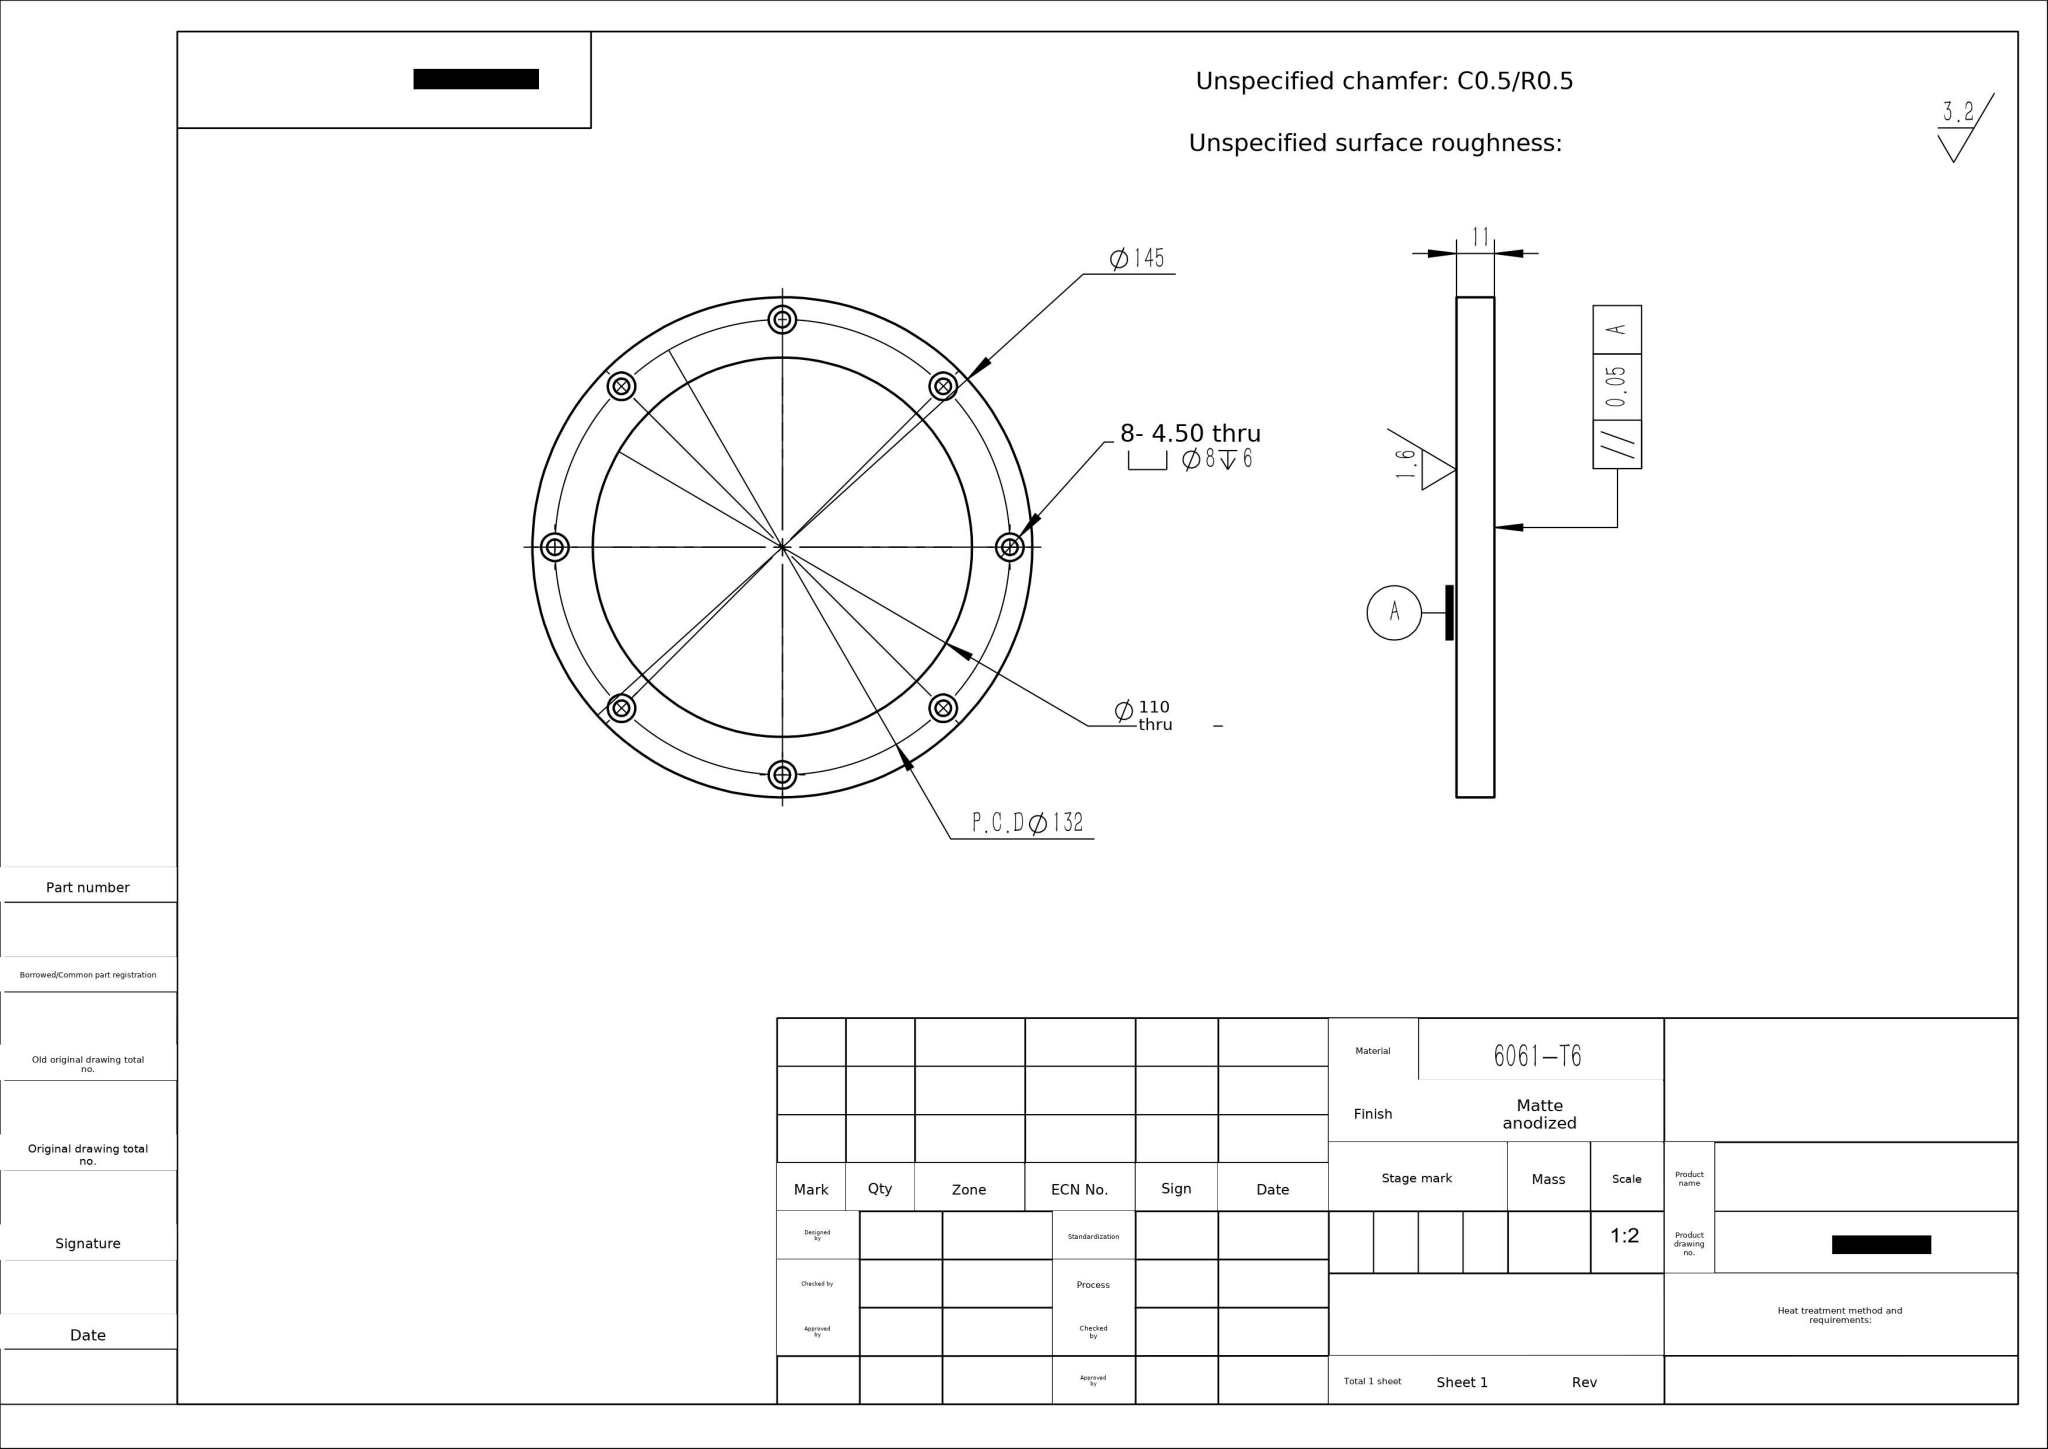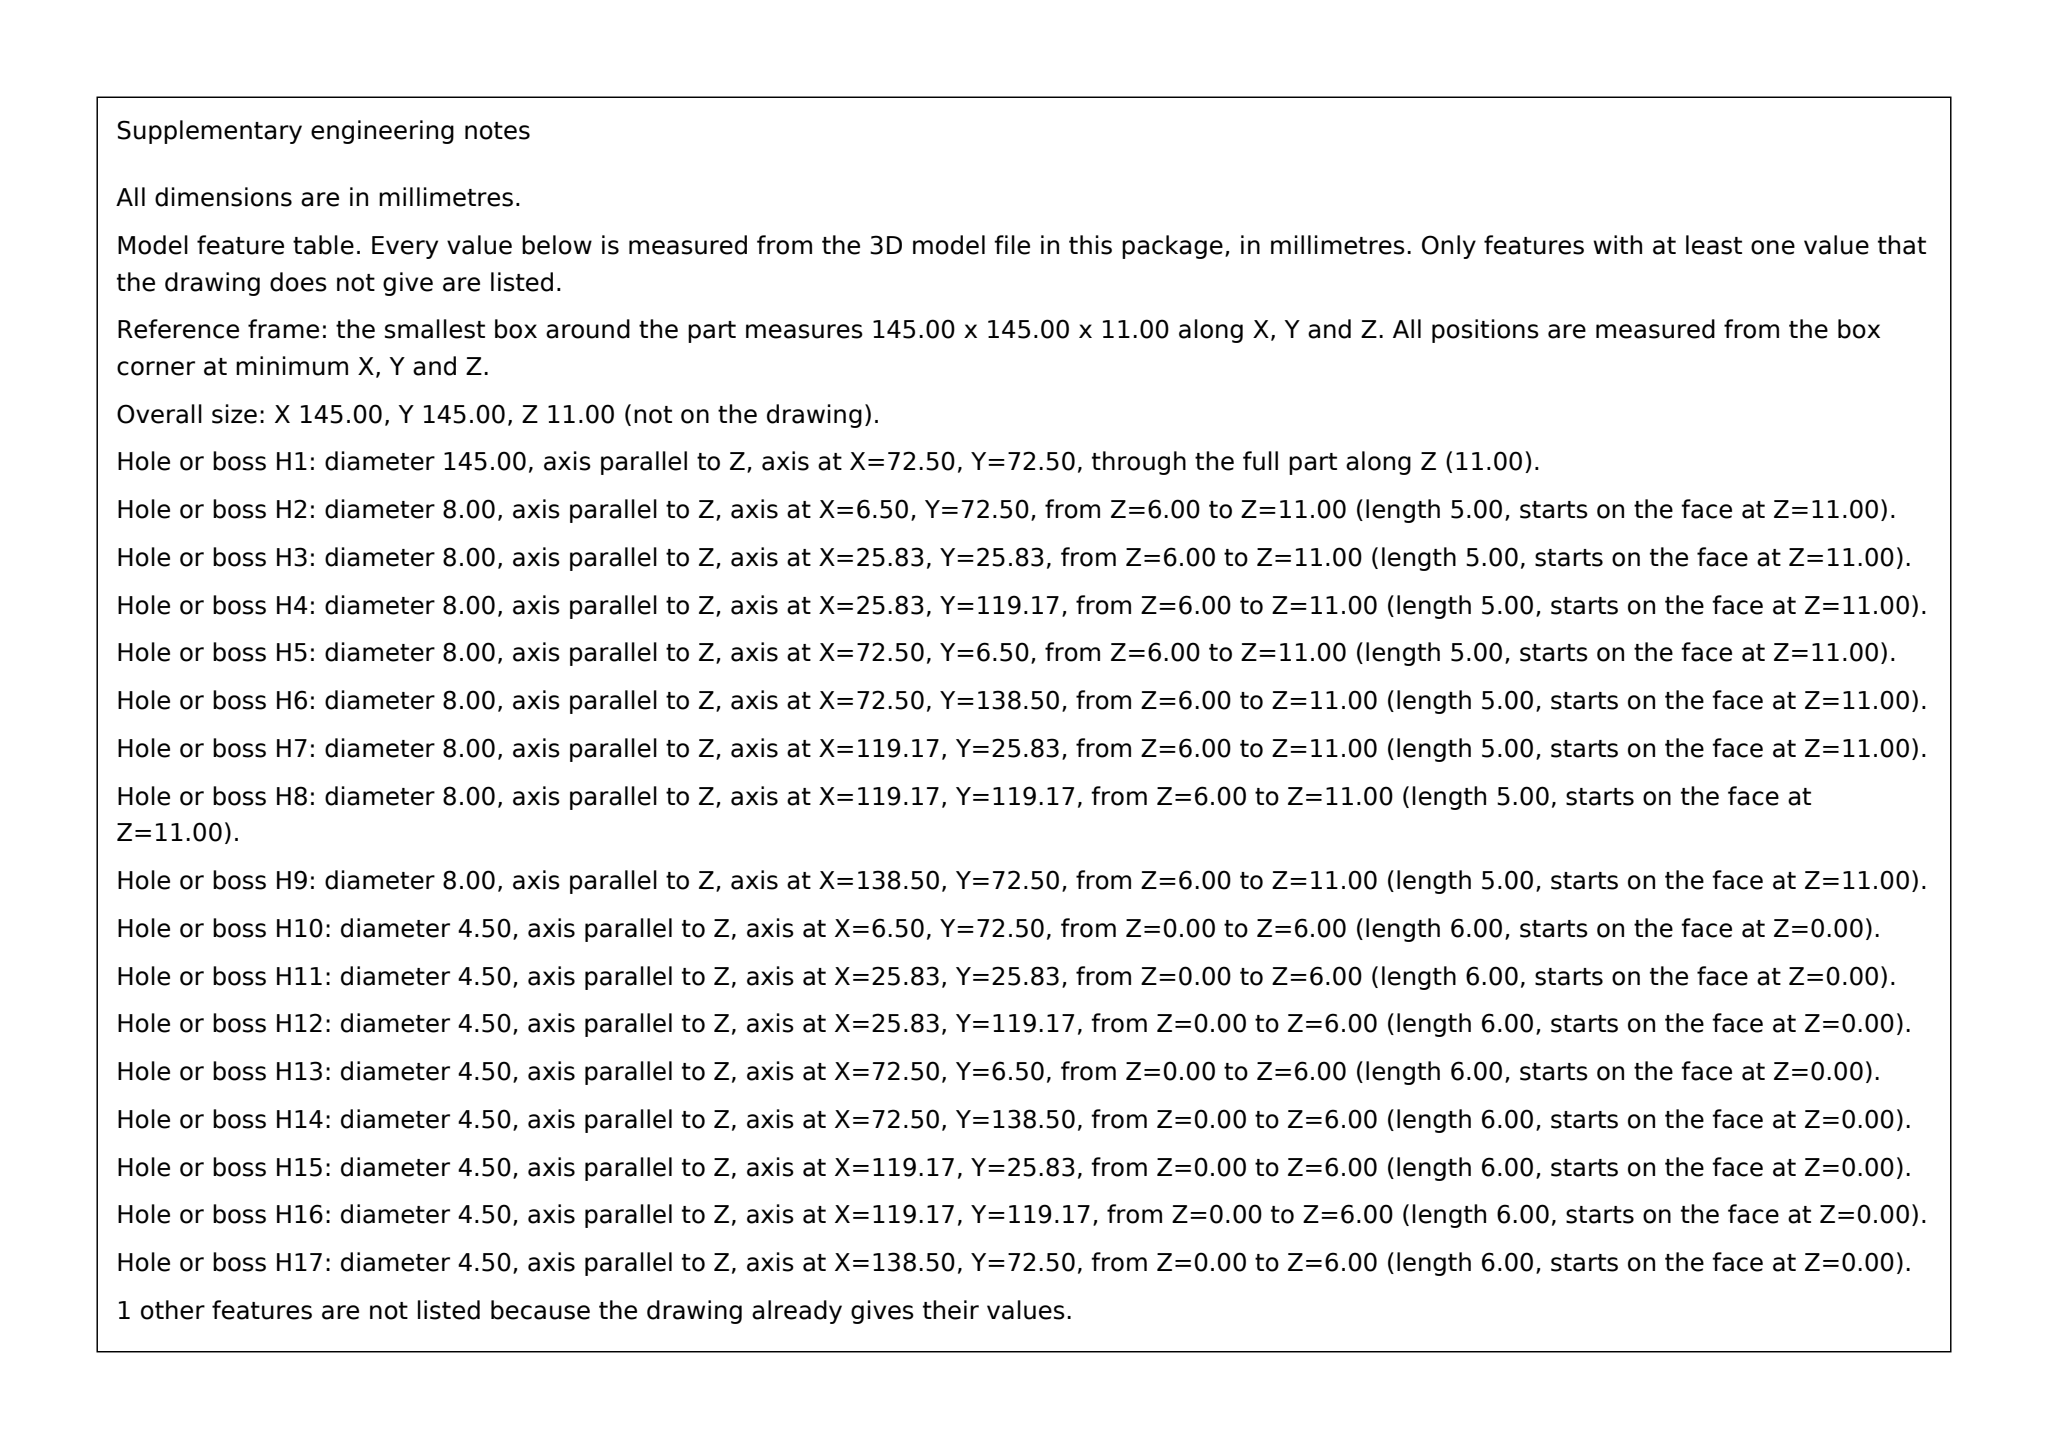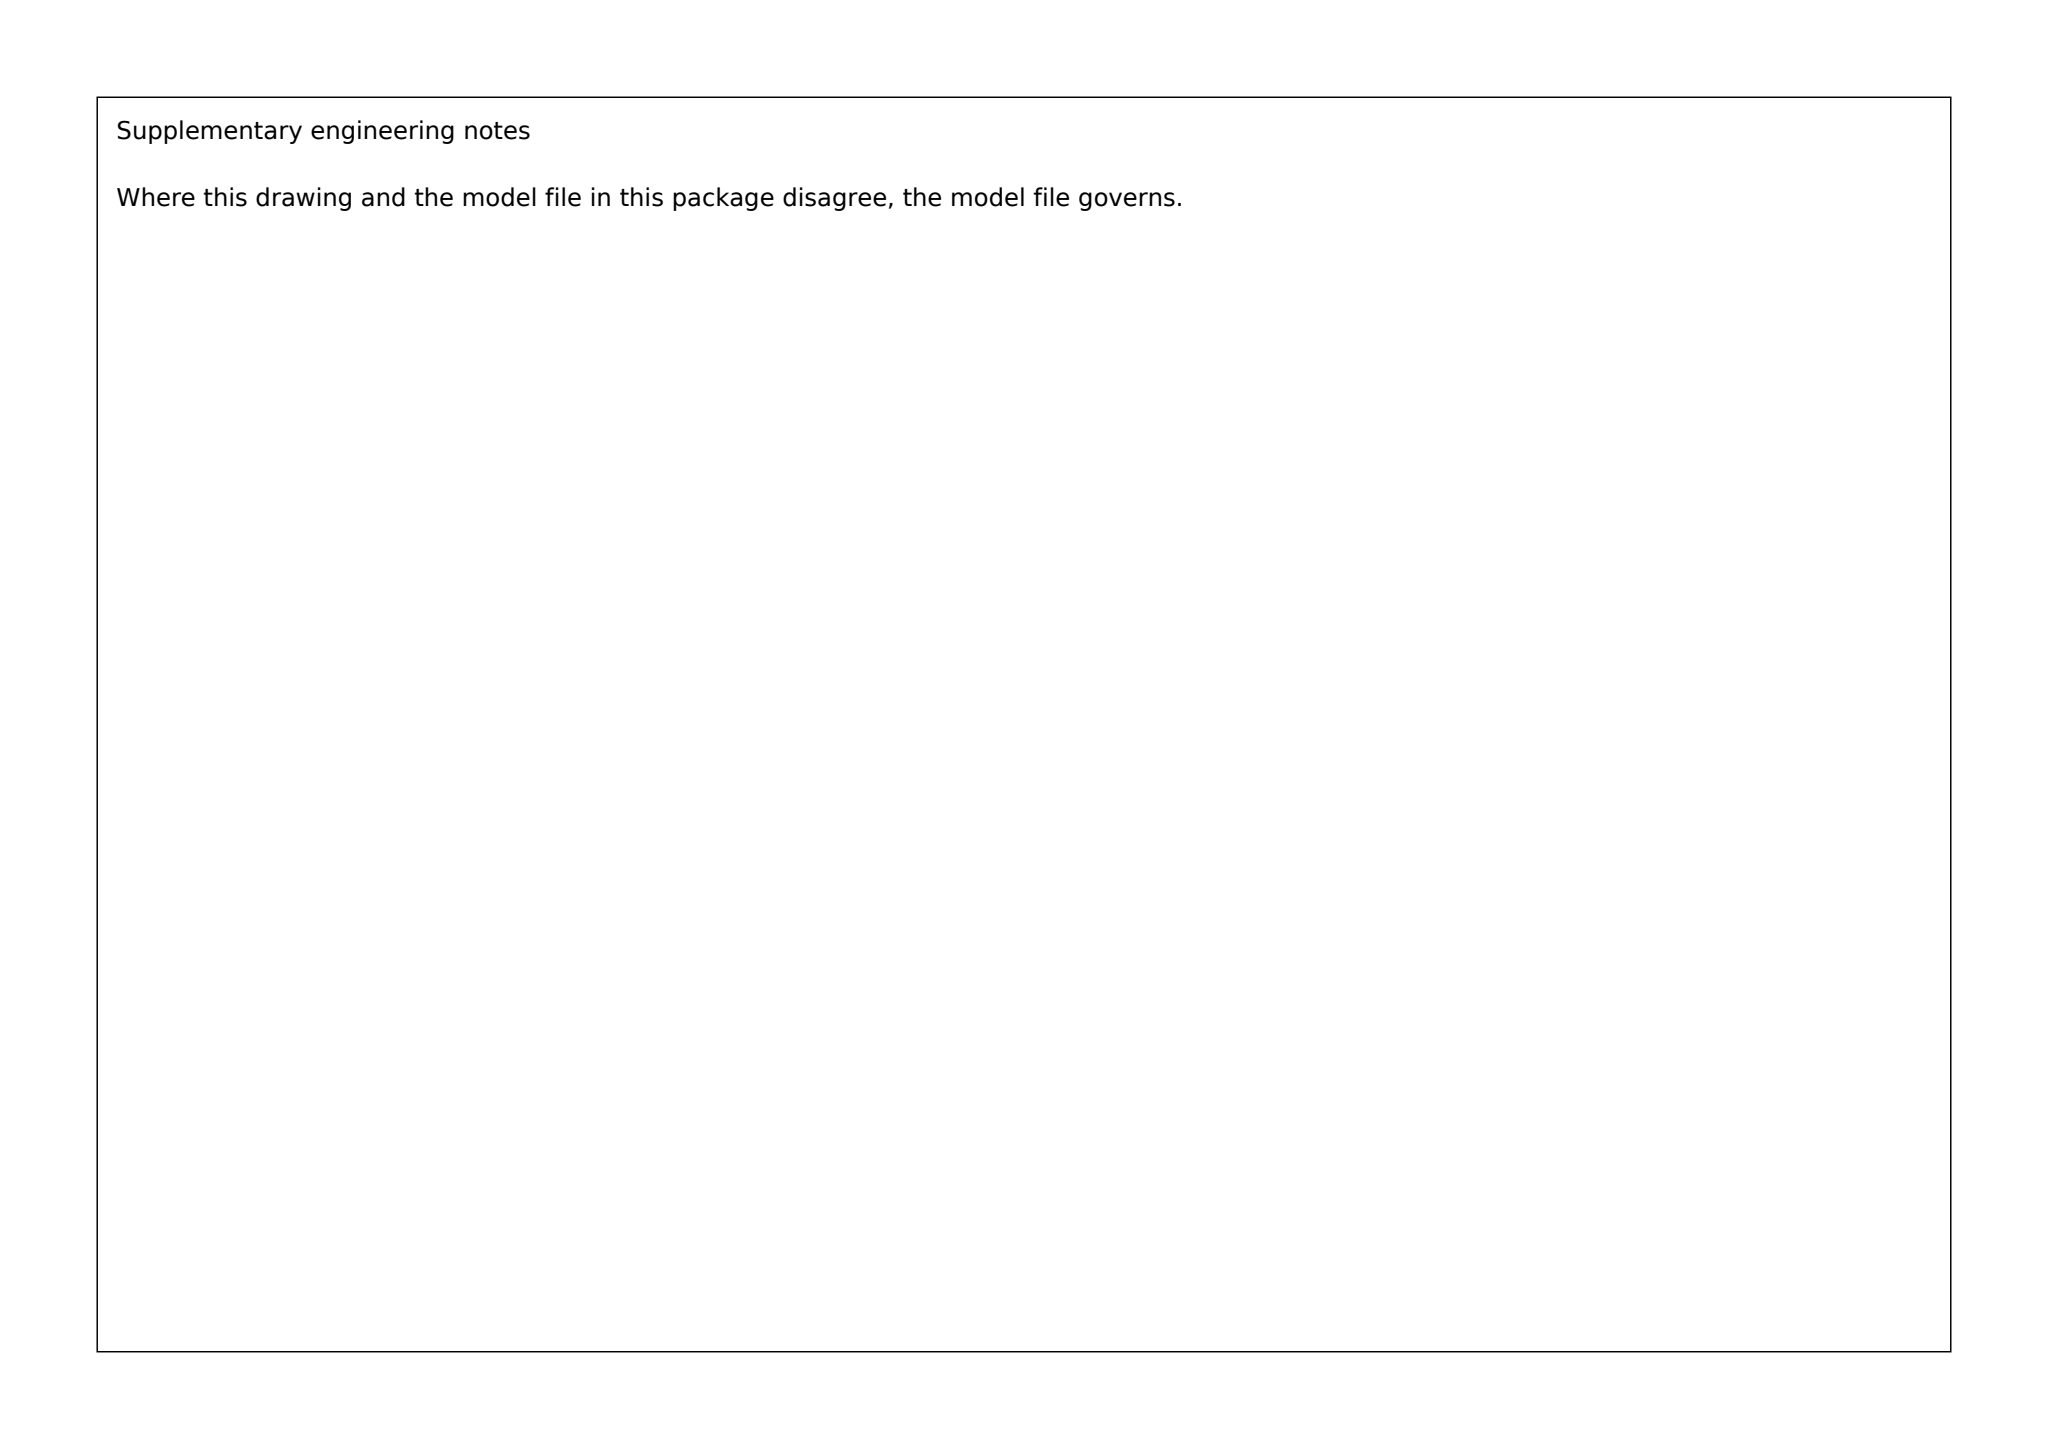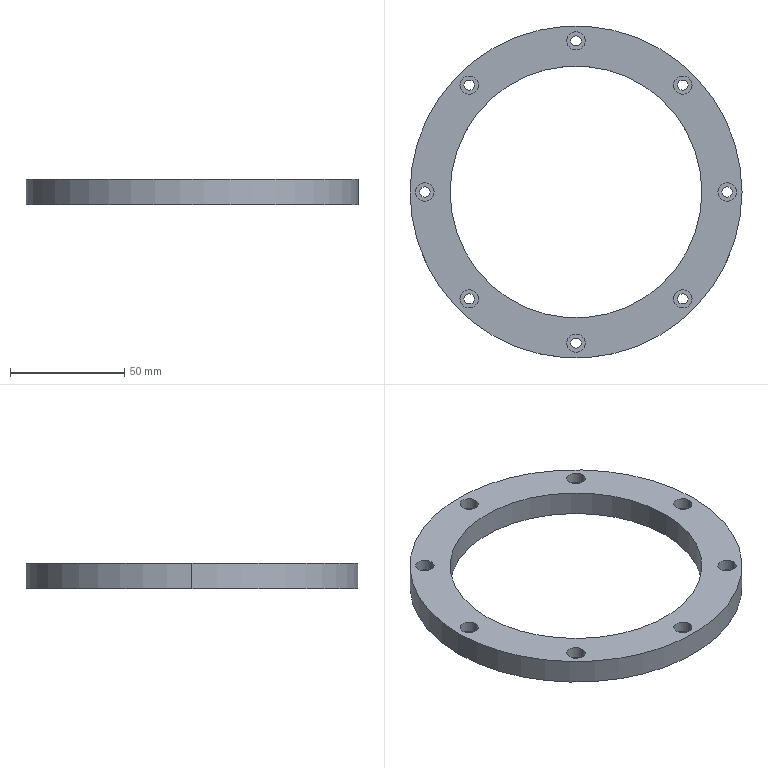Part | SolidWorks | mm | material 6061-T6 | 1 solid | 46 faces | box 145 x 145 x 11 mm | volume 74332 mm3 | cylinder 36 | plane 10 | commonest cylinder face diameters 8 x16 4.5 x16 110 x2 145 x2
build123d program:
from build123d import *

# Parameters (mm, degrees)
SKETCH1_R           = 72.5
SKETCH1_R_2         = 55
BOSS_EXTRUDE1_DEPTH = 11
SKETCH2_R           = 2.25
CUT_EXTRUDE1_DEPTH  = 104.119
SKETCH3_R           = 4
CUT_EXTRUDE2_DEPTH  = 5


with BuildPart() as part:
    # Sketch1 → Boss-Extrude1 (new body)
    with BuildSketch(Plane.XY):
        Circle(SKETCH1_R)
        Circle(SKETCH1_R_2, mode=Mode.SUBTRACT)
    extrude(amount=BOSS_EXTRUDE1_DEPTH)

    # Sketch2 → Cut-Extrude1 (cut, through all)
    with BuildSketch(Plane.XY.offset(11)):
        with Locations((0, 66)):
            Circle(SKETCH2_R)
        with Locations((46.669, 46.669)):
            Circle(SKETCH2_R)
        with Locations((66, 0)):
            Circle(SKETCH2_R)
        with Locations((46.669, -46.669)):
            Circle(SKETCH2_R)
        with Locations((0, -66)):
            Circle(SKETCH2_R)
        with Locations((-46.669, -46.669)):
            Circle(SKETCH2_R)
        with Locations((-66, 0)):
            Circle(SKETCH2_R)
        with Locations((-46.669, 46.669)):
            Circle(SKETCH2_R)
    extrude(amount=-CUT_EXTRUDE1_DEPTH, mode=Mode.SUBTRACT)

    # Sketch3 → Cut-Extrude2 (cut)
    with BuildSketch(Plane.XY.offset(11)):
        with Locations((46.669, 46.669)):
            Circle(SKETCH3_R)
        with Locations((66, 0)):
            Circle(SKETCH3_R)
        with Locations((46.669, -46.669)):
            Circle(SKETCH3_R)
        with Locations((0, -66)):
            Circle(SKETCH3_R)
        with Locations((-46.669, -46.669)):
            Circle(SKETCH3_R)
        with Locations((-66, 0)):
            Circle(SKETCH3_R)
        with Locations((-46.669, 46.669)):
            Circle(SKETCH3_R)
        with Locations((0, 66)):
            Circle(SKETCH3_R)
    extrude(amount=-CUT_EXTRUDE2_DEPTH, mode=Mode.SUBTRACT)


solid = part.part